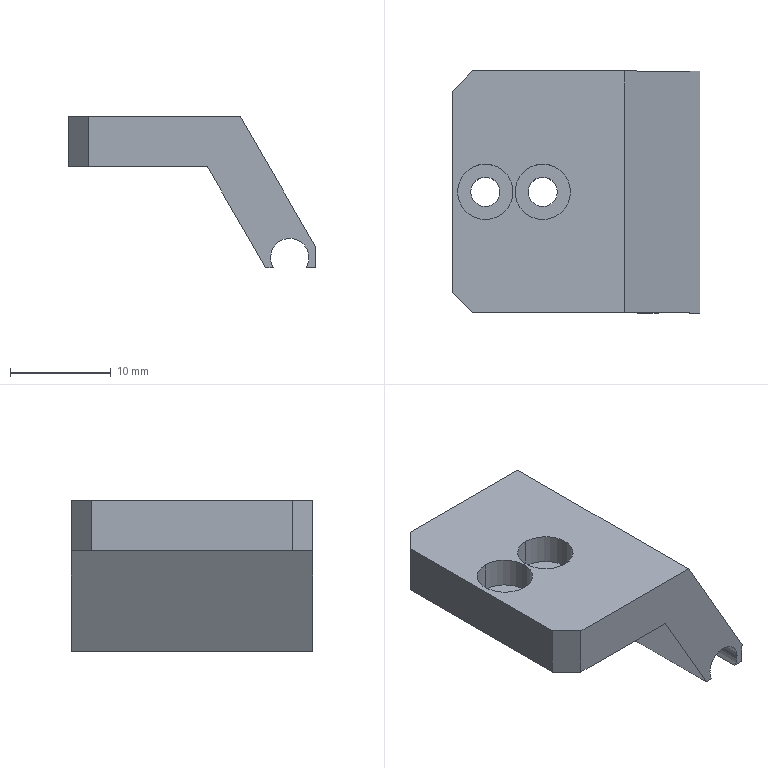Component | SolidWorks | 31298300012MechanicalFinger-1 | 1 solid | 25 faces | box 24.6 x 24 x 15 mm | volume 3262 mm3 | plane 14 | cylinder 11 | commonest cylinder face diameters 5.5 x4 2.9 x4 3.8 x3 | material Q235-A
build123d program:
from build123d import *

# Parameters (mm, degrees)
BOSS_EXTRUDE1_DEPTH                               = 12
M2_5_HEX_SOCKET_HEAD_CAP_SCREW_CBORE1_D           = 2.9
M2_5_HEX_SOCKET_HEAD_CAP_SCREW_CBORE1_CBORE_D     = 5.5
M2_5_HEX_SOCKET_HEAD_CAP_SCREW_CBORE1_CBORE_DEPTH = 3
CHAMFER1_SIZE                                     = 2
SKETCH5_R                                         = 1.9
CUT_EXTRUDE2_DEPTH                                = 38.499


with BuildPart() as part:
    # Sketch1 → Boss-Extrude1 (new, symmetric)
    with BuildSketch(Plane.XY):
        Polygon((0, 0), (17.094, 0), (24.6, -13), (24.6, -15), (19.6, -15), (13.826, -5), (0, -5), align=None)
    extrude(amount=BOSS_EXTRUDE1_DEPTH, both=True)

    # M2.5 Hex Socket Head Cap Screw CBORE1 (through all)
    with Locations(Plane(origin=(0, 0, 0), x_dir=(-1, 0, 0), z_dir=(0, 1, 0))):
        with Locations((-3.3, 0), (-9, 0)):
            CounterBoreHole(M2_5_HEX_SOCKET_HEAD_CAP_SCREW_CBORE1_D / 2, M2_5_HEX_SOCKET_HEAD_CAP_SCREW_CBORE1_CBORE_D / 2, M2_5_HEX_SOCKET_HEAD_CAP_SCREW_CBORE1_CBORE_DEPTH)

    # Chamfer1
    chamfer1_edges = [part.edges().sort_by_distance(p)[0] for p in [
        (0, -2.5, 12),
        (0, -2.5, -12),
    ]]
    chamfer(chamfer1_edges, length=CHAMFER1_SIZE)

    # Sketch5 → Cut-Extrude2 (cut, through all)
    with BuildSketch(Plane.XY.offset(12)):
        with Locations((22, -14)):
            Circle(SKETCH5_R)
    extrude(amount=-CUT_EXTRUDE2_DEPTH, mode=Mode.SUBTRACT)


solid = part.part

# Placed as in the assembly
solid = solid.moved(Location((188.87, 43.668, 52.929), (90, 0, 0)))
STEP:
#1=COLOUR_RGB('',0.7922,0.8196,0.9333);
#2=FILL_AREA_STYLE_COLOUR('',#1);
#3=FILL_AREA_STYLE('',(#2));
#4=SURFACE_STYLE_FILL_AREA(#3);
#5=SURFACE_SIDE_STYLE('',(#4));
#6=SURFACE_STYLE_USAGE(.BOTH.,#5);
#7=PRESENTATION_STYLE_ASSIGNMENT((#6));
#8=CARTESIAN_POINT('',(8.238,2.192,1.493));
#9=VERTEX_POINT('',#8);
#10=CARTESIAN_POINT('',(8.227,2.192,1.533));
#11=VERTEX_POINT('',#10);
#12=CARTESIAN_POINT('',(8.302,2.192,1.533));
#13=DIRECTION('',(-0.,1.,-0.));
#14=DIRECTION('',(-1.,0.,0.));
#15=AXIS2_PLACEMENT_3D('',#12,#13,#14);
#16=CIRCLE('',#15,0.0748);
#17=EDGE_CURVE('',#9,#11,#16,.T.);
#18=ORIENTED_EDGE('',*,*,#17,.T.);
#19=CARTESIAN_POINT('',(8.227,1.247,1.533));
#20=VERTEX_POINT('',#19);
#21=CARTESIAN_POINT('',(8.227,2.192,1.533));
#22=DIRECTION('',(0.,-1.,0.));
#23=VECTOR('',#22,39.37);
#24=LINE('',#21,#23);
#25=EDGE_CURVE('',#11,#20,#24,.T.);
#26=ORIENTED_EDGE('',*,*,#25,.T.);
#27=CARTESIAN_POINT('',(8.238,1.247,1.493));
#28=VERTEX_POINT('',#27);
#29=CARTESIAN_POINT('',(8.302,1.247,1.533));
#30=DIRECTION('',(0.,-1.,0.));
#31=DIRECTION('',(1.,0.,0.));
#32=AXIS2_PLACEMENT_3D('',#29,#30,#31);
#33=CIRCLE('',#32,0.0748);
#34=EDGE_CURVE('',#20,#28,#33,.T.);
#35=ORIENTED_EDGE('',*,*,#34,.T.);
#36=CARTESIAN_POINT('',(8.238,2.192,1.493));
#37=DIRECTION('',(0.,-1.,0.));
#38=VECTOR('',#37,39.37);
#39=LINE('',#36,#38);
#40=EDGE_CURVE('',#9,#28,#39,.T.);
#41=ORIENTED_EDGE('',*,*,#40,.F.);
#42=EDGE_LOOP('',(#18,#26,#35,#41));
#43=FACE_OUTER_BOUND('',#42,.T.);
#44=CARTESIAN_POINT('',(8.302,2.192,1.533));
#45=DIRECTION('',(0.,-1.,0.));
#46=DIRECTION('',(1.,0.,0.));
#47=AXIS2_PLACEMENT_3D('',#44,#45,#46);
#48=CYLINDRICAL_SURFACE('',#47,0.0748);
#49=ADVANCED_FACE('',(#43),#48,.F.);
#50=ORIENTED_EDGE('',*,*,#25,.F.);
#51=CARTESIAN_POINT('',(8.377,2.192,1.533));
#52=VERTEX_POINT('',#51);
#53=CARTESIAN_POINT('',(8.302,2.192,1.533));
#54=DIRECTION('',(-0.,1.,-0.));
#55=DIRECTION('',(-1.,0.,0.));
#56=AXIS2_PLACEMENT_3D('',#53,#54,#55);
#57=CIRCLE('',#56,0.0748);
#58=EDGE_CURVE('',#11,#52,#57,.T.);
#59=ORIENTED_EDGE('',*,*,#58,.T.);
#60=CARTESIAN_POINT('',(8.377,1.247,1.533));
#61=VERTEX_POINT('',#60);
#62=CARTESIAN_POINT('',(8.377,2.192,1.533));
#63=DIRECTION('',(0.,-1.,0.));
#64=VECTOR('',#63,39.37);
#65=LINE('',#62,#64);
#66=EDGE_CURVE('',#52,#61,#65,.T.);
#67=ORIENTED_EDGE('',*,*,#66,.T.);
#68=CARTESIAN_POINT('',(8.302,1.247,1.533));
#69=DIRECTION('',(0.,-1.,0.));
#70=DIRECTION('',(1.,0.,0.));
#71=AXIS2_PLACEMENT_3D('',#68,#69,#70);
#72=CIRCLE('',#71,0.0748);
#73=EDGE_CURVE('',#61,#20,#72,.T.);
#74=ORIENTED_EDGE('',*,*,#73,.T.);
#75=EDGE_LOOP('',(#50,#59,#67,#74));
#76=FACE_OUTER_BOUND('',#75,.T.);
#77=CARTESIAN_POINT('',(8.302,2.192,1.533));
#78=DIRECTION('',(0.,-1.,0.));
#79=DIRECTION('',(1.,0.,0.));
#80=AXIS2_PLACEMENT_3D('',#77,#78,#79);
#81=CYLINDRICAL_SURFACE('',#80,0.0748);
#82=ADVANCED_FACE('',(#76),#81,.F.);
#83=CARTESIAN_POINT('',(7.566,1.827,1.966));
#84=VERTEX_POINT('',#83);
#85=CARTESIAN_POINT('',(7.566,1.611,1.966));
#86=VERTEX_POINT('',#85);
#87=CARTESIAN_POINT('',(7.566,1.719,1.966));
#88=DIRECTION('',(0.,0.,1.));
#89=DIRECTION('',(0.,-1.,0.));
#90=AXIS2_PLACEMENT_3D('',#87,#88,#89);
#91=CIRCLE('',#90,0.1083);
#92=EDGE_CURVE('',#84,#86,#91,.T.);
#93=ORIENTED_EDGE('',*,*,#92,.F.);
#94=CARTESIAN_POINT('',(7.566,1.827,2.084));
#95=VERTEX_POINT('',#94);
#96=CARTESIAN_POINT('',(7.566,1.827,2.084));
#97=DIRECTION('',(0.,0.,1.));
#98=VECTOR('',#97,39.37);
#99=LINE('',#96,#98);
#100=EDGE_CURVE('',#84,#95,#99,.T.);
#101=ORIENTED_EDGE('',*,*,#100,.T.);
#102=CARTESIAN_POINT('',(7.566,1.611,2.084));
#103=VERTEX_POINT('',#102);
#104=CARTESIAN_POINT('',(7.566,1.719,2.084));
#105=DIRECTION('',(0.,0.,1.));
#106=DIRECTION('',(0.,-1.,0.));
#107=AXIS2_PLACEMENT_3D('',#104,#105,#106);
#108=CIRCLE('',#107,0.1083);
#109=EDGE_CURVE('',#95,#103,#108,.T.);
#110=ORIENTED_EDGE('',*,*,#109,.T.);
#111=CARTESIAN_POINT('',(7.566,1.611,2.084));
#112=DIRECTION('',(0.,0.,1.));
#113=VECTOR('',#112,39.37);
#114=LINE('',#111,#113);
#115=EDGE_CURVE('',#86,#103,#114,.T.);
#116=ORIENTED_EDGE('',*,*,#115,.F.);
#117=EDGE_LOOP('',(#93,#101,#110,#116));
#118=FACE_OUTER_BOUND('',#117,.T.);
#119=CARTESIAN_POINT('',(7.566,1.719,2.084));
#120=DIRECTION('',(0.,0.,1.));
#121=DIRECTION('',(0.,-1.,0.));
#122=AXIS2_PLACEMENT_3D('',#119,#120,#121);
#123=CYLINDRICAL_SURFACE('',#122,0.1083);
#124=ADVANCED_FACE('',(#118),#123,.F.);
#125=CARTESIAN_POINT('',(7.566,1.776,1.887));
#126=VERTEX_POINT('',#125);
#127=CARTESIAN_POINT('',(7.566,1.662,1.887));
#128=VERTEX_POINT('',#127);
#129=CARTESIAN_POINT('',(7.566,1.719,1.887));
#130=DIRECTION('',(0.,0.,1.));
#131=DIRECTION('',(-1.,0.,0.));
#132=AXIS2_PLACEMENT_3D('',#129,#130,#131);
#133=CIRCLE('',#132,0.05709);
#134=EDGE_CURVE('',#126,#128,#133,.T.);
#135=ORIENTED_EDGE('',*,*,#134,.F.);
#136=CARTESIAN_POINT('',(7.566,1.776,1.966));
#137=VERTEX_POINT('',#136);
#138=CARTESIAN_POINT('',(7.566,1.776,2.084));
#139=DIRECTION('',(0.,0.,1.));
#140=VECTOR('',#139,39.37);
#141=LINE('',#138,#140);
#142=EDGE_CURVE('',#126,#137,#141,.T.);
#143=ORIENTED_EDGE('',*,*,#142,.T.);
#144=CARTESIAN_POINT('',(7.566,1.662,1.966));
#145=VERTEX_POINT('',#144);
#146=CARTESIAN_POINT('',(7.566,1.719,1.966));
#147=DIRECTION('',(0.,0.,1.));
#148=DIRECTION('',(0.,-1.,0.));
#149=AXIS2_PLACEMENT_3D('',#146,#147,#148);
#150=CIRCLE('',#149,0.05709);
#151=EDGE_CURVE('',#137,#145,#150,.T.);
#152=ORIENTED_EDGE('',*,*,#151,.T.);
#153=CARTESIAN_POINT('',(7.566,1.662,2.084));
#154=DIRECTION('',(0.,0.,1.));
#155=VECTOR('',#154,39.37);
#156=LINE('',#153,#155);
#157=EDGE_CURVE('',#128,#145,#156,.T.);
#158=ORIENTED_EDGE('',*,*,#157,.F.);
#159=EDGE_LOOP('',(#135,#143,#152,#158));
#160=FACE_OUTER_BOUND('',#159,.T.);
#161=CARTESIAN_POINT('',(7.566,1.719,2.084));
#162=DIRECTION('',(0.,0.,1.));
#163=DIRECTION('',(0.,-1.,0.));
#164=AXIS2_PLACEMENT_3D('',#161,#162,#163);
#165=CYLINDRICAL_SURFACE('',#164,0.05709);
#166=ADVANCED_FACE('',(#160),#165,.F.);
#167=CARTESIAN_POINT('',(7.79,1.827,1.966));
#168=VERTEX_POINT('',#167);
#169=CARTESIAN_POINT('',(7.79,1.611,1.966));
#170=VERTEX_POINT('',#169);
#171=CARTESIAN_POINT('',(7.79,1.719,1.966));
#172=DIRECTION('',(0.,0.,1.));
#173=DIRECTION('',(0.,-1.,0.));
#174=AXIS2_PLACEMENT_3D('',#171,#172,#173);
#175=CIRCLE('',#174,0.1083);
#176=EDGE_CURVE('',#168,#170,#175,.T.);
#177=ORIENTED_EDGE('',*,*,#176,.F.);
#178=CARTESIAN_POINT('',(7.79,1.827,2.084));
#179=VERTEX_POINT('',#178);
#180=CARTESIAN_POINT('',(7.79,1.827,2.084));
#181=DIRECTION('',(0.,0.,1.));
#182=VECTOR('',#181,39.37);
#183=LINE('',#180,#182);
#184=EDGE_CURVE('',#168,#179,#183,.T.);
#185=ORIENTED_EDGE('',*,*,#184,.T.);
#186=CARTESIAN_POINT('',(7.79,1.611,2.084));
#187=VERTEX_POINT('',#186);
#188=CARTESIAN_POINT('',(7.79,1.719,2.084));
#189=DIRECTION('',(0.,0.,1.));
#190=DIRECTION('',(0.,-1.,0.));
#191=AXIS2_PLACEMENT_3D('',#188,#189,#190);
#192=CIRCLE('',#191,0.1083);
#193=EDGE_CURVE('',#179,#187,#192,.T.);
#194=ORIENTED_EDGE('',*,*,#193,.T.);
#195=CARTESIAN_POINT('',(7.79,1.611,2.084));
#196=DIRECTION('',(0.,0.,1.));
#197=VECTOR('',#196,39.37);
#198=LINE('',#195,#197);
#199=EDGE_CURVE('',#170,#187,#198,.T.);
#200=ORIENTED_EDGE('',*,*,#199,.F.);
#201=EDGE_LOOP('',(#177,#185,#194,#200));
#202=FACE_OUTER_BOUND('',#201,.T.);
#203=CARTESIAN_POINT('',(7.79,1.719,2.084));
#204=DIRECTION('',(0.,0.,1.));
#205=DIRECTION('',(0.,-1.,0.));
#206=AXIS2_PLACEMENT_3D('',#203,#204,#205);
#207=CYLINDRICAL_SURFACE('',#206,0.1083);
#208=ADVANCED_FACE('',(#202),#207,.F.);
#209=CARTESIAN_POINT('',(7.79,1.776,1.887));
#210=VERTEX_POINT('',#209);
#211=CARTESIAN_POINT('',(7.79,1.662,1.887));
#212=VERTEX_POINT('',#211);
#213=CARTESIAN_POINT('',(7.79,1.719,1.887));
#214=DIRECTION('',(0.,0.,1.));
#215=DIRECTION('',(-1.,0.,0.));
#216=AXIS2_PLACEMENT_3D('',#213,#214,#215);
#217=CIRCLE('',#216,0.05709);
#218=EDGE_CURVE('',#210,#212,#217,.T.);
#219=ORIENTED_EDGE('',*,*,#218,.F.);
#220=CARTESIAN_POINT('',(7.79,1.776,1.966));
#221=VERTEX_POINT('',#220);
#222=CARTESIAN_POINT('',(7.79,1.776,2.084));
#223=DIRECTION('',(0.,0.,1.));
#224=VECTOR('',#223,39.37);
#225=LINE('',#222,#224);
#226=EDGE_CURVE('',#210,#221,#225,.T.);
#227=ORIENTED_EDGE('',*,*,#226,.T.);
#228=CARTESIAN_POINT('',(7.79,1.662,1.966));
#229=VERTEX_POINT('',#228);
#230=CARTESIAN_POINT('',(7.79,1.719,1.966));
#231=DIRECTION('',(0.,0.,1.));
#232=DIRECTION('',(0.,-1.,0.));
#233=AXIS2_PLACEMENT_3D('',#230,#231,#232);
#234=CIRCLE('',#233,0.05709);
#235=EDGE_CURVE('',#221,#229,#234,.T.);
#236=ORIENTED_EDGE('',*,*,#235,.T.);
#237=CARTESIAN_POINT('',(7.79,1.662,2.084));
#238=DIRECTION('',(0.,0.,1.));
#239=VECTOR('',#238,39.37);
#240=LINE('',#237,#239);
#241=EDGE_CURVE('',#212,#229,#240,.T.);
#242=ORIENTED_EDGE('',*,*,#241,.F.);
#243=EDGE_LOOP('',(#219,#227,#236,#242));
#244=FACE_OUTER_BOUND('',#243,.T.);
#245=CARTESIAN_POINT('',(7.79,1.719,2.084));
#246=DIRECTION('',(0.,0.,1.));
#247=DIRECTION('',(0.,-1.,0.));
#248=AXIS2_PLACEMENT_3D('',#245,#246,#247);
#249=CYLINDRICAL_SURFACE('',#248,0.05709);
#250=ADVANCED_FACE('',(#244),#249,.F.);
#251=CARTESIAN_POINT('',(8.207,2.192,1.493));
#252=VERTEX_POINT('',#251);
#253=CARTESIAN_POINT('',(8.404,2.192,1.493));
#254=DIRECTION('',(1.,0.,-0.));
#255=VECTOR('',#254,39.37);
#256=LINE('',#253,#255);
#257=EDGE_CURVE('',#252,#9,#256,.T.);
#258=ORIENTED_EDGE('',*,*,#257,.T.);
#259=ORIENTED_EDGE('',*,*,#40,.T.);
#260=CARTESIAN_POINT('',(8.207,1.247,1.493));
#261=VERTEX_POINT('',#260);
#262=CARTESIAN_POINT('',(8.404,1.247,1.493));
#263=DIRECTION('',(1.,0.,-0.));
#264=VECTOR('',#263,39.37);
#265=LINE('',#262,#264);
#266=EDGE_CURVE('',#261,#28,#265,.T.);
#267=ORIENTED_EDGE('',*,*,#266,.F.);
#268=CARTESIAN_POINT('',(8.207,1.247,1.493));
#269=DIRECTION('',(-0.,1.,-0.));
#270=VECTOR('',#269,39.37);
#271=LINE('',#268,#270);
#272=EDGE_CURVE('',#261,#252,#271,.T.);
#273=ORIENTED_EDGE('',*,*,#272,.T.);
#274=EDGE_LOOP('',(#258,#259,#267,#273));
#275=FACE_OUTER_BOUND('',#274,.T.);
#276=CARTESIAN_POINT('',(8.404,1.247,1.493));
#277=DIRECTION('',(0.,0.,1.));
#278=DIRECTION('',(0.,-1.,0.));
#279=AXIS2_PLACEMENT_3D('',#276,#277,#278);
#280=PLANE('',#279);
#281=ADVANCED_FACE('',(#275),#280,.F.);
#282=CARTESIAN_POINT('',(7.436,1.326,1.887));
#283=VERTEX_POINT('',#282);
#284=CARTESIAN_POINT('',(7.436,2.113,1.887));
#285=VERTEX_POINT('',#284);
#286=CARTESIAN_POINT('',(7.436,1.247,1.887));
#287=DIRECTION('',(-0.,1.,-0.));
#288=VECTOR('',#287,39.37);
#289=LINE('',#286,#288);
#290=EDGE_CURVE('',#283,#285,#289,.T.);
#291=ORIENTED_EDGE('',*,*,#290,.F.);
#292=CARTESIAN_POINT('',(7.436,1.326,2.084));
#293=VERTEX_POINT('',#292);
#294=CARTESIAN_POINT('',(7.436,1.326,1.887));
#295=DIRECTION('',(0.,0.,1.));
#296=VECTOR('',#295,39.37);
#297=LINE('',#294,#296);
#298=EDGE_CURVE('',#283,#293,#297,.T.);
#299=ORIENTED_EDGE('',*,*,#298,.T.);
#300=CARTESIAN_POINT('',(7.436,2.113,2.084));
#301=VERTEX_POINT('',#300);
#302=CARTESIAN_POINT('',(7.436,1.247,2.084));
#303=DIRECTION('',(-0.,1.,-0.));
#304=VECTOR('',#303,39.37);
#305=LINE('',#302,#304);
#306=EDGE_CURVE('',#293,#301,#305,.T.);
#307=ORIENTED_EDGE('',*,*,#306,.T.);
#308=CARTESIAN_POINT('',(7.436,2.113,1.887));
#309=DIRECTION('',(-0.,-0.,-1.));
#310=VECTOR('',#309,39.37);
#311=LINE('',#308,#310);
#312=EDGE_CURVE('',#301,#285,#311,.T.);
#313=ORIENTED_EDGE('',*,*,#312,.T.);
#314=EDGE_LOOP('',(#291,#299,#307,#313));
#315=FACE_OUTER_BOUND('',#314,.T.);
#316=CARTESIAN_POINT('',(7.436,1.247,1.887));
#317=DIRECTION('',(1.,0.,-0.));
#318=DIRECTION('',(-0.,1.,-0.));
#319=AXIS2_PLACEMENT_3D('',#316,#317,#318);
#320=PLANE('',#319);
#321=ADVANCED_FACE('',(#315),#320,.F.);
#322=CARTESIAN_POINT('',(7.566,1.719,1.887));
#323=DIRECTION('',(0.,0.,1.));
#324=DIRECTION('',(-1.,0.,0.));
#325=AXIS2_PLACEMENT_3D('',#322,#323,#324);
#326=CIRCLE('',#325,0.05709);
#327=EDGE_CURVE('',#128,#126,#326,.T.);
#328=ORIENTED_EDGE('',*,*,#327,.T.);
#329=ORIENTED_EDGE('',*,*,#134,.T.);
#330=EDGE_LOOP('',(#328,#329));
#331=FACE_BOUND('',#330,.T.);
#332=CARTESIAN_POINT('',(7.79,1.719,1.887));
#333=DIRECTION('',(0.,0.,1.));
#334=DIRECTION('',(-1.,0.,0.));
#335=AXIS2_PLACEMENT_3D('',#332,#333,#334);
#336=CIRCLE('',#335,0.05709);
#337=EDGE_CURVE('',#212,#210,#336,.T.);
#338=ORIENTED_EDGE('',*,*,#337,.T.);
#339=ORIENTED_EDGE('',*,*,#218,.T.);
#340=EDGE_LOOP('',(#338,#339));
#341=FACE_BOUND('',#340,.T.);
#342=CARTESIAN_POINT('',(7.515,1.247,1.887));
#343=VERTEX_POINT('',#342);
#344=CARTESIAN_POINT('',(7.98,1.247,1.887));
#345=VERTEX_POINT('',#344);
#346=CARTESIAN_POINT('',(7.98,1.247,1.887));
#347=DIRECTION('',(1.,0.,-0.));
#348=VECTOR('',#347,39.37);
#349=LINE('',#346,#348);
#350=EDGE_CURVE('',#343,#345,#349,.T.);
#351=ORIENTED_EDGE('',*,*,#350,.F.);
#352=CARTESIAN_POINT('',(7.515,1.247,1.887));
#353=DIRECTION('',(-0.7071,0.7071,0.));
#354=VECTOR('',#353,39.37);
#355=LINE('',#352,#354);
#356=EDGE_CURVE('',#343,#283,#355,.T.);
#357=ORIENTED_EDGE('',*,*,#356,.T.);
#358=ORIENTED_EDGE('',*,*,#290,.T.);
#359=CARTESIAN_POINT('',(7.515,2.192,1.887));
#360=VERTEX_POINT('',#359);
#361=CARTESIAN_POINT('',(7.436,2.113,1.887));
#362=DIRECTION('',(0.7071,0.7071,-0.));
#363=VECTOR('',#362,39.37);
#364=LINE('',#361,#363);
#365=EDGE_CURVE('',#285,#360,#364,.T.);
#366=ORIENTED_EDGE('',*,*,#365,.T.);
#367=CARTESIAN_POINT('',(7.98,2.192,1.887));
#368=VERTEX_POINT('',#367);
#369=CARTESIAN_POINT('',(7.98,2.192,1.887));
#370=DIRECTION('',(1.,0.,-0.));
#371=VECTOR('',#370,39.37);
#372=LINE('',#369,#371);
#373=EDGE_CURVE('',#360,#368,#372,.T.);
#374=ORIENTED_EDGE('',*,*,#373,.T.);
#375=CARTESIAN_POINT('',(7.98,1.247,1.887));
#376=DIRECTION('',(-0.,1.,-0.));
#377=VECTOR('',#376,39.37);
#378=LINE('',#375,#377);
#379=EDGE_CURVE('',#345,#368,#378,.T.);
#380=ORIENTED_EDGE('',*,*,#379,.F.);
#381=EDGE_LOOP('',(#351,#357,#358,#366,#374,#380));
#382=FACE_OUTER_BOUND('',#381,.T.);
#383=CARTESIAN_POINT('',(7.98,1.247,1.887));
#384=DIRECTION('',(0.,0.,1.));
#385=DIRECTION('',(-1.,-0.,0.));
#386=AXIS2_PLACEMENT_3D('',#383,#384,#385);
#387=PLANE('',#386);
#388=ADVANCED_FACE('',(#331,#341,#382),#387,.F.);
#389=CARTESIAN_POINT('',(8.207,2.192,1.493));
#390=DIRECTION('',(0.5,0.,-0.866));
#391=VECTOR('',#390,39.37);
#392=LINE('',#389,#391);
#393=EDGE_CURVE('',#368,#252,#392,.T.);
#394=ORIENTED_EDGE('',*,*,#393,.T.);
#395=ORIENTED_EDGE('',*,*,#272,.F.);
#396=CARTESIAN_POINT('',(8.207,1.247,1.493));
#397=DIRECTION('',(0.5,0.,-0.866));
#398=VECTOR('',#397,39.37);
#399=LINE('',#396,#398);
#400=EDGE_CURVE('',#345,#261,#399,.T.);
#401=ORIENTED_EDGE('',*,*,#400,.F.);
#402=ORIENTED_EDGE('',*,*,#379,.T.);
#403=EDGE_LOOP('',(#394,#395,#401,#402));
#404=FACE_OUTER_BOUND('',#403,.T.);
#405=CARTESIAN_POINT('',(8.207,1.247,1.493));
#406=DIRECTION('',(0.866,0.,0.5));
#407=DIRECTION('',(-0.5,-0.,0.866));
#408=AXIS2_PLACEMENT_3D('',#405,#406,#407);
#409=PLANE('',#408);
#410=ADVANCED_FACE('',(#404),#409,.F.);
#411=CARTESIAN_POINT('',(8.366,1.247,1.493));
#412=VERTEX_POINT('',#411);
#413=CARTESIAN_POINT('',(8.404,1.247,1.493));
#414=VERTEX_POINT('',#413);
#415=CARTESIAN_POINT('',(8.404,1.247,1.493));
#416=DIRECTION('',(1.,0.,-0.));
#417=VECTOR('',#416,39.37);
#418=LINE('',#415,#417);
#419=EDGE_CURVE('',#412,#414,#418,.T.);
#420=ORIENTED_EDGE('',*,*,#419,.F.);
#421=CARTESIAN_POINT('',(8.366,2.192,1.493));
#422=VERTEX_POINT('',#421);
#423=CARTESIAN_POINT('',(8.366,2.192,1.493));
#424=DIRECTION('',(-0.,1.,-0.));
#425=VECTOR('',#424,39.37);
#426=LINE('',#423,#425);
#427=EDGE_CURVE('',#412,#422,#426,.T.);
#428=ORIENTED_EDGE('',*,*,#427,.T.);
#429=CARTESIAN_POINT('',(8.404,2.192,1.493));
#430=VERTEX_POINT('',#429);
#431=CARTESIAN_POINT('',(8.404,2.192,1.493));
#432=DIRECTION('',(1.,0.,-0.));
#433=VECTOR('',#432,39.37);
#434=LINE('',#431,#433);
#435=EDGE_CURVE('',#422,#430,#434,.T.);
#436=ORIENTED_EDGE('',*,*,#435,.T.);
#437=CARTESIAN_POINT('',(8.404,1.247,1.493));
#438=DIRECTION('',(-0.,1.,-0.));
#439=VECTOR('',#438,39.37);
#440=LINE('',#437,#439);
#441=EDGE_CURVE('',#414,#430,#440,.T.);
#442=ORIENTED_EDGE('',*,*,#441,.F.);
#443=EDGE_LOOP('',(#420,#428,#436,#442));
#444=FACE_OUTER_BOUND('',#443,.T.);
#445=CARTESIAN_POINT('',(8.404,1.247,1.493));
#446=DIRECTION('',(0.,0.,1.));
#447=DIRECTION('',(0.,-1.,0.));
#448=AXIS2_PLACEMENT_3D('',#445,#446,#447);
#449=PLANE('',#448);
#450=ADVANCED_FACE('',(#444),#449,.F.);
#451=CARTESIAN_POINT('',(8.404,2.192,1.572));
#452=VERTEX_POINT('',#451);
#453=CARTESIAN_POINT('',(8.404,2.192,1.572));
#454=DIRECTION('',(0.,0.,1.));
#455=VECTOR('',#454,39.37);
#456=LINE('',#453,#455);
#457=EDGE_CURVE('',#430,#452,#456,.T.);
#458=ORIENTED_EDGE('',*,*,#457,.T.);
#459=CARTESIAN_POINT('',(8.404,1.247,1.572));
#460=VERTEX_POINT('',#459);
#461=CARTESIAN_POINT('',(8.404,1.247,1.572));
#462=DIRECTION('',(-0.,1.,-0.));
#463=VECTOR('',#462,39.37);
#464=LINE('',#461,#463);
#465=EDGE_CURVE('',#460,#452,#464,.T.);
#466=ORIENTED_EDGE('',*,*,#465,.F.);
#467=CARTESIAN_POINT('',(8.404,1.247,1.572));
#468=DIRECTION('',(0.,0.,1.));
#469=VECTOR('',#468,39.37);
#470=LINE('',#467,#469);
#471=EDGE_CURVE('',#414,#460,#470,.T.);
#472=ORIENTED_EDGE('',*,*,#471,.F.);
#473=ORIENTED_EDGE('',*,*,#441,.T.);
#474=EDGE_LOOP('',(#458,#466,#472,#473));
#475=FACE_OUTER_BOUND('',#474,.T.);
#476=CARTESIAN_POINT('',(8.404,1.247,1.572));
#477=DIRECTION('',(-1.,-0.,0.));
#478=DIRECTION('',(0.,-1.,0.));
#479=AXIS2_PLACEMENT_3D('',#476,#477,#478);
#480=PLANE('',#479);
#481=ADVANCED_FACE('',(#475),#480,.F.);
#482=CARTESIAN_POINT('',(8.109,2.192,2.084));
#483=VERTEX_POINT('',#482);
#484=CARTESIAN_POINT('',(8.109,2.192,2.084));
#485=DIRECTION('',(-0.5,-0.,0.866));
#486=VECTOR('',#485,39.37);
#487=LINE('',#484,#486);
#488=EDGE_CURVE('',#452,#483,#487,.T.);
#489=ORIENTED_EDGE('',*,*,#488,.T.);
#490=CARTESIAN_POINT('',(8.109,1.247,2.084));
#491=VERTEX_POINT('',#490);
#492=CARTESIAN_POINT('',(8.109,1.247,2.084));
#493=DIRECTION('',(-0.,1.,-0.));
#494=VECTOR('',#493,39.37);
#495=LINE('',#492,#494);
#496=EDGE_CURVE('',#491,#483,#495,.T.);
#497=ORIENTED_EDGE('',*,*,#496,.F.);
#498=CARTESIAN_POINT('',(8.109,1.247,2.084));
#499=DIRECTION('',(-0.5,-0.,0.866));
#500=VECTOR('',#499,39.37);
#501=LINE('',#498,#500);
#502=EDGE_CURVE('',#460,#491,#501,.T.);
#503=ORIENTED_EDGE('',*,*,#502,.F.);
#504=ORIENTED_EDGE('',*,*,#465,.T.);
#505=EDGE_LOOP('',(#489,#497,#503,#504));
#506=FACE_OUTER_BOUND('',#505,.T.);
#507=CARTESIAN_POINT('',(8.109,1.247,2.084));
#508=DIRECTION('',(-0.866,-0.,-0.5));
#509=DIRECTION('',(0.5,0.,-0.866));
#510=AXIS2_PLACEMENT_3D('',#507,#508,#509);
#511=PLANE('',#510);
#512=ADVANCED_FACE('',(#506),#511,.F.);
#513=CARTESIAN_POINT('',(7.566,1.719,2.084));
#514=DIRECTION('',(0.,0.,1.));
#515=DIRECTION('',(0.,-1.,0.));
#516=AXIS2_PLACEMENT_3D('',#513,#514,#515);
#517=CIRCLE('',#516,0.1083);
#518=EDGE_CURVE('',#103,#95,#517,.T.);
#519=ORIENTED_EDGE('',*,*,#518,.F.);
#520=ORIENTED_EDGE('',*,*,#109,.F.);
#521=EDGE_LOOP('',(#519,#520));
#522=FACE_BOUND('',#521,.T.);
#523=CARTESIAN_POINT('',(7.79,1.719,2.084));
#524=DIRECTION('',(0.,0.,1.));
#525=DIRECTION('',(0.,-1.,0.));
#526=AXIS2_PLACEMENT_3D('',#523,#524,#525);
#527=CIRCLE('',#526,0.1083);
#528=EDGE_CURVE('',#187,#179,#527,.T.);
#529=ORIENTED_EDGE('',*,*,#528,.F.);
#530=ORIENTED_EDGE('',*,*,#193,.F.);
#531=EDGE_LOOP('',(#529,#530));
#532=FACE_BOUND('',#531,.T.);
#533=ORIENTED_EDGE('',*,*,#306,.F.);
#534=CARTESIAN_POINT('',(7.515,1.247,2.084));
#535=VERTEX_POINT('',#534);
#536=CARTESIAN_POINT('',(7.515,1.247,2.084));
#537=DIRECTION('',(0.7071,-0.7071,-0.));
#538=VECTOR('',#537,39.37);
#539=LINE('',#536,#538);
#540=EDGE_CURVE('',#293,#535,#539,.T.);
#541=ORIENTED_EDGE('',*,*,#540,.T.);
#542=CARTESIAN_POINT('',(7.436,1.247,2.084));
#543=DIRECTION('',(-1.,-0.,0.));
#544=VECTOR('',#543,39.37);
#545=LINE('',#542,#544);
#546=EDGE_CURVE('',#491,#535,#545,.T.);
#547=ORIENTED_EDGE('',*,*,#546,.F.);
#548=ORIENTED_EDGE('',*,*,#496,.T.);
#549=CARTESIAN_POINT('',(7.515,2.192,2.084));
#550=VERTEX_POINT('',#549);
#551=CARTESIAN_POINT('',(7.436,2.192,2.084));
#552=DIRECTION('',(-1.,-0.,0.));
#553=VECTOR('',#552,39.37);
#554=LINE('',#551,#553);
#555=EDGE_CURVE('',#483,#550,#554,.T.);
#556=ORIENTED_EDGE('',*,*,#555,.T.);
#557=CARTESIAN_POINT('',(7.436,2.113,2.084));
#558=DIRECTION('',(-0.7071,-0.7071,0.));
#559=VECTOR('',#558,39.37);
#560=LINE('',#557,#559);
#561=EDGE_CURVE('',#550,#301,#560,.T.);
#562=ORIENTED_EDGE('',*,*,#561,.T.);
#563=EDGE_LOOP('',(#533,#541,#547,#548,#556,#562));
#564=FACE_OUTER_BOUND('',#563,.T.);
#565=CARTESIAN_POINT('',(7.436,1.247,2.084));
#566=DIRECTION('',(-0.,-0.,-1.));
#567=DIRECTION('',(-0.,1.,-0.));
#568=AXIS2_PLACEMENT_3D('',#565,#566,#567);
#569=PLANE('',#568);
#570=ADVANCED_FACE('',(#522,#532,#564),#569,.F.);
#571=ORIENTED_EDGE('',*,*,#266,.T.);
#572=ORIENTED_EDGE('',*,*,#34,.F.);
#573=ORIENTED_EDGE('',*,*,#73,.F.);
#574=CARTESIAN_POINT('',(8.302,1.247,1.533));
#575=DIRECTION('',(0.,-1.,0.));
#576=DIRECTION('',(1.,0.,0.));
#577=AXIS2_PLACEMENT_3D('',#574,#575,#576);
#578=CIRCLE('',#577,0.0748);
#579=EDGE_CURVE('',#412,#61,#578,.T.);
#580=ORIENTED_EDGE('',*,*,#579,.F.);
#581=ORIENTED_EDGE('',*,*,#419,.T.);
#582=ORIENTED_EDGE('',*,*,#471,.T.);
#583=ORIENTED_EDGE('',*,*,#502,.T.);
#584=ORIENTED_EDGE('',*,*,#546,.T.);
#585=CARTESIAN_POINT('',(7.515,1.247,2.084));
#586=DIRECTION('',(-0.,-0.,-1.));
#587=VECTOR('',#586,39.37);
#588=LINE('',#585,#587);
#589=EDGE_CURVE('',#535,#343,#588,.T.);
#590=ORIENTED_EDGE('',*,*,#589,.T.);
#591=ORIENTED_EDGE('',*,*,#350,.T.);
#592=ORIENTED_EDGE('',*,*,#400,.T.);
#593=EDGE_LOOP('',(#571,#572,#573,#580,#581,#582,#583,#584,#590,#591,#592));
#594=FACE_OUTER_BOUND('',#593,.T.);
#595=CARTESIAN_POINT('',(7.436,1.247,2.084));
#596=DIRECTION('',(-0.,1.,-0.));
#597=DIRECTION('',(-1.,-0.,0.));
#598=AXIS2_PLACEMENT_3D('',#595,#596,#597);
#599=PLANE('',#598);
#600=ADVANCED_FACE('',(#594),#599,.F.);
#601=ORIENTED_EDGE('',*,*,#17,.F.);
#602=ORIENTED_EDGE('',*,*,#257,.F.);
#603=ORIENTED_EDGE('',*,*,#393,.F.);
#604=ORIENTED_EDGE('',*,*,#373,.F.);
#605=CARTESIAN_POINT('',(7.515,2.192,2.084));
#606=DIRECTION('',(0.,0.,1.));
#607=VECTOR('',#606,39.37);
#608=LINE('',#605,#607);
#609=EDGE_CURVE('',#360,#550,#608,.T.);
#610=ORIENTED_EDGE('',*,*,#609,.T.);
#611=ORIENTED_EDGE('',*,*,#555,.F.);
#612=ORIENTED_EDGE('',*,*,#488,.F.);
#613=ORIENTED_EDGE('',*,*,#457,.F.);
#614=ORIENTED_EDGE('',*,*,#435,.F.);
#615=CARTESIAN_POINT('',(8.302,2.192,1.533));
#616=DIRECTION('',(-0.,1.,-0.));
#617=DIRECTION('',(-1.,0.,0.));
#618=AXIS2_PLACEMENT_3D('',#615,#616,#617);
#619=CIRCLE('',#618,0.0748);
#620=EDGE_CURVE('',#52,#422,#619,.T.);
#621=ORIENTED_EDGE('',*,*,#620,.F.);
#622=ORIENTED_EDGE('',*,*,#58,.F.);
#623=EDGE_LOOP('',(#601,#602,#603,#604,#610,#611,#612,#613,#614,#621,#622));
#624=FACE_OUTER_BOUND('',#623,.T.);
#625=CARTESIAN_POINT('',(7.436,2.192,2.084));
#626=DIRECTION('',(-0.,1.,-0.));
#627=DIRECTION('',(-1.,-0.,0.));
#628=AXIS2_PLACEMENT_3D('',#625,#626,#627);
#629=PLANE('',#628);
#630=ADVANCED_FACE('',(#624),#629,.T.);
#631=ORIENTED_EDGE('',*,*,#226,.F.);
#632=ORIENTED_EDGE('',*,*,#337,.F.);
#633=ORIENTED_EDGE('',*,*,#241,.T.);
#634=CARTESIAN_POINT('',(7.79,1.719,1.966));
#635=DIRECTION('',(0.,0.,1.));
#636=DIRECTION('',(0.,-1.,0.));
#637=AXIS2_PLACEMENT_3D('',#634,#635,#636);
#638=CIRCLE('',#637,0.05709);
#639=EDGE_CURVE('',#229,#221,#638,.T.);
#640=ORIENTED_EDGE('',*,*,#639,.T.);
#641=EDGE_LOOP('',(#631,#632,#633,#640));
#642=FACE_OUTER_BOUND('',#641,.T.);
#643=CARTESIAN_POINT('',(7.79,1.719,2.084));
#644=DIRECTION('',(0.,0.,1.));
#645=DIRECTION('',(0.,-1.,0.));
#646=AXIS2_PLACEMENT_3D('',#643,#644,#645);
#647=CYLINDRICAL_SURFACE('',#646,0.05709);
#648=ADVANCED_FACE('',(#642),#647,.F.);
#649=ORIENTED_EDGE('',*,*,#639,.F.);
#650=ORIENTED_EDGE('',*,*,#235,.F.);
#651=EDGE_LOOP('',(#649,#650));
#652=FACE_BOUND('',#651,.T.);
#653=CARTESIAN_POINT('',(7.79,1.719,1.966));
#654=DIRECTION('',(0.,0.,1.));
#655=DIRECTION('',(0.,-1.,0.));
#656=AXIS2_PLACEMENT_3D('',#653,#654,#655);
#657=CIRCLE('',#656,0.1083);
#658=EDGE_CURVE('',#170,#168,#657,.T.);
#659=ORIENTED_EDGE('',*,*,#658,.T.);
#660=ORIENTED_EDGE('',*,*,#176,.T.);
#661=EDGE_LOOP('',(#659,#660));
#662=FACE_OUTER_BOUND('',#661,.T.);
#663=CARTESIAN_POINT('',(7.847,1.719,1.966));
#664=DIRECTION('',(-0.,-0.,-1.));
#665=DIRECTION('',(-0.,1.,-0.));
#666=AXIS2_PLACEMENT_3D('',#663,#664,#665);
#667=PLANE('',#666);
#668=ADVANCED_FACE('',(#652,#662),#667,.F.);
#669=ORIENTED_EDGE('',*,*,#184,.F.);
#670=ORIENTED_EDGE('',*,*,#658,.F.);
#671=ORIENTED_EDGE('',*,*,#199,.T.);
#672=ORIENTED_EDGE('',*,*,#528,.T.);
#673=EDGE_LOOP('',(#669,#670,#671,#672));
#674=FACE_OUTER_BOUND('',#673,.T.);
#675=CARTESIAN_POINT('',(7.79,1.719,2.084));
#676=DIRECTION('',(0.,0.,1.));
#677=DIRECTION('',(0.,-1.,0.));
#678=AXIS2_PLACEMENT_3D('',#675,#676,#677);
#679=CYLINDRICAL_SURFACE('',#678,0.1083);
#680=ADVANCED_FACE('',(#674),#679,.F.);
#681=ORIENTED_EDGE('',*,*,#142,.F.);
#682=ORIENTED_EDGE('',*,*,#327,.F.);
#683=ORIENTED_EDGE('',*,*,#157,.T.);
#684=CARTESIAN_POINT('',(7.566,1.719,1.966));
#685=DIRECTION('',(0.,0.,1.));
#686=DIRECTION('',(0.,-1.,0.));
#687=AXIS2_PLACEMENT_3D('',#684,#685,#686);
#688=CIRCLE('',#687,0.05709);
#689=EDGE_CURVE('',#145,#137,#688,.T.);
#690=ORIENTED_EDGE('',*,*,#689,.T.);
#691=EDGE_LOOP('',(#681,#682,#683,#690));
#692=FACE_OUTER_BOUND('',#691,.T.);
#693=CARTESIAN_POINT('',(7.566,1.719,2.084));
#694=DIRECTION('',(0.,0.,1.));
#695=DIRECTION('',(0.,-1.,0.));
#696=AXIS2_PLACEMENT_3D('',#693,#694,#695);
#697=CYLINDRICAL_SURFACE('',#696,0.05709);
#698=ADVANCED_FACE('',(#692),#697,.F.);
#699=ORIENTED_EDGE('',*,*,#689,.F.);
#700=ORIENTED_EDGE('',*,*,#151,.F.);
#701=EDGE_LOOP('',(#699,#700));
#702=FACE_BOUND('',#701,.T.);
#703=CARTESIAN_POINT('',(7.566,1.719,1.966));
#704=DIRECTION('',(0.,0.,1.));
#705=DIRECTION('',(0.,-1.,0.));
#706=AXIS2_PLACEMENT_3D('',#703,#704,#705);
#707=CIRCLE('',#706,0.1083);
#708=EDGE_CURVE('',#86,#84,#707,.T.);
#709=ORIENTED_EDGE('',*,*,#708,.T.);
#710=ORIENTED_EDGE('',*,*,#92,.T.);
#711=EDGE_LOOP('',(#709,#710));
#712=FACE_OUTER_BOUND('',#711,.T.);
#713=CARTESIAN_POINT('',(7.623,1.719,1.966));
#714=DIRECTION('',(-0.,-0.,-1.));
#715=DIRECTION('',(-0.,1.,-0.));
#716=AXIS2_PLACEMENT_3D('',#713,#714,#715);
#717=PLANE('',#716);
#718=ADVANCED_FACE('',(#702,#712),#717,.F.);
#719=ORIENTED_EDGE('',*,*,#100,.F.);
#720=ORIENTED_EDGE('',*,*,#708,.F.);
#721=ORIENTED_EDGE('',*,*,#115,.T.);
#722=ORIENTED_EDGE('',*,*,#518,.T.);
#723=EDGE_LOOP('',(#719,#720,#721,#722));
#724=FACE_OUTER_BOUND('',#723,.T.);
#725=CARTESIAN_POINT('',(7.566,1.719,2.084));
#726=DIRECTION('',(0.,0.,1.));
#727=DIRECTION('',(0.,-1.,0.));
#728=AXIS2_PLACEMENT_3D('',#725,#726,#727);
#729=CYLINDRICAL_SURFACE('',#728,0.1083);
#730=ADVANCED_FACE('',(#724),#729,.F.);
#731=ORIENTED_EDGE('',*,*,#540,.F.);
#732=ORIENTED_EDGE('',*,*,#298,.F.);
#733=ORIENTED_EDGE('',*,*,#356,.F.);
#734=ORIENTED_EDGE('',*,*,#589,.F.);
#735=EDGE_LOOP('',(#731,#732,#733,#734));
#736=FACE_OUTER_BOUND('',#735,.T.);
#737=CARTESIAN_POINT('',(7.515,1.247,2.084));
#738=DIRECTION('',(0.7071,0.7071,-0.));
#739=DIRECTION('',(-0.7071,0.7071,0.));
#740=AXIS2_PLACEMENT_3D('',#737,#738,#739);
#741=PLANE('',#740);
#742=ADVANCED_FACE('',(#736),#741,.F.);
#743=ORIENTED_EDGE('',*,*,#561,.F.);
#744=ORIENTED_EDGE('',*,*,#609,.F.);
#745=ORIENTED_EDGE('',*,*,#365,.F.);
#746=ORIENTED_EDGE('',*,*,#312,.F.);
#747=EDGE_LOOP('',(#743,#744,#745,#746));
#748=FACE_OUTER_BOUND('',#747,.T.);
#749=CARTESIAN_POINT('',(7.436,2.113,1.887));
#750=DIRECTION('',(-0.7071,0.7071,0.));
#751=DIRECTION('',(-0.7071,-0.7071,0.));
#752=AXIS2_PLACEMENT_3D('',#749,#750,#751);
#753=PLANE('',#752);
#754=ADVANCED_FACE('',(#748),#753,.T.);
#755=ORIENTED_EDGE('',*,*,#66,.F.);
#756=ORIENTED_EDGE('',*,*,#620,.T.);
#757=ORIENTED_EDGE('',*,*,#427,.F.);
#758=ORIENTED_EDGE('',*,*,#579,.T.);
#759=EDGE_LOOP('',(#755,#756,#757,#758));
#760=FACE_OUTER_BOUND('',#759,.T.);
#761=CARTESIAN_POINT('',(8.302,2.192,1.533));
#762=DIRECTION('',(0.,-1.,0.));
#763=DIRECTION('',(1.,0.,0.));
#764=AXIS2_PLACEMENT_3D('',#761,#762,#763);
#765=CYLINDRICAL_SURFACE('',#764,0.0748);
#766=ADVANCED_FACE('',(#760),#765,.F.);
#767=CLOSED_SHELL('',(#49,#82,#124,#166,#208,#250,#281,#321,#388,#410,#450,#481,#512,#570,#600,#630,#648,#668,#680,#698,#718,#730,#742,#754,#766));
#768=MANIFOLD_SOLID_BREP('',#767);
#769=STYLED_ITEM('',(#7),#768);
#770=(LENGTH_UNIT()NAMED_UNIT(*)SI_UNIT($,.METRE.));
#771=LENGTH_MEASURE_WITH_UNIT(LENGTH_MEASURE(0.0254),#770);
#772=DIMENSIONAL_EXPONENTS(1.,0.,0.,0.,0.,0.,0.);
#773=(CONVERSION_BASED_UNIT('',#771)LENGTH_UNIT()NAMED_UNIT(#772));
#774=UNCERTAINTY_MEASURE_WITH_UNIT(LENGTH_MEASURE(0.00001),#773,'','');
#775=(NAMED_UNIT(*)PLANE_ANGLE_UNIT()SI_UNIT($,.RADIAN.));
#776=(NAMED_UNIT(*)SI_UNIT($,.STERADIAN.)SOLID_ANGLE_UNIT());
#777=(GEOMETRIC_REPRESENTATION_CONTEXT(3)GLOBAL_UNCERTAINTY_ASSIGNED_CONTEXT((#774))GLOBAL_UNIT_ASSIGNED_CONTEXT((#773,#775,#776))REPRESENTATION_CONTEXT('',''));
#778=MECHANICAL_DESIGN_GEOMETRIC_PRESENTATION_REPRESENTATION('',(#769),#777);
#779=CARTESIAN_POINT('',(0.,0.,0.));
#780=DIRECTION('',(0.,0.,1.));
#781=DIRECTION('',(1.,0.,0.));
#782=AXIS2_PLACEMENT_3D('',#779,#780,#781);
#783=(LENGTH_UNIT()NAMED_UNIT(*)SI_UNIT($,.METRE.));
#784=LENGTH_MEASURE_WITH_UNIT(LENGTH_MEASURE(0.0254),#783);
#785=DIMENSIONAL_EXPONENTS(1.,0.,0.,0.,0.,0.,0.);
#786=(CONVERSION_BASED_UNIT('',#784)LENGTH_UNIT()NAMED_UNIT(#785));
#787=UNCERTAINTY_MEASURE_WITH_UNIT(LENGTH_MEASURE(0.00001),#786,'','');
#788=(NAMED_UNIT(*)PLANE_ANGLE_UNIT()SI_UNIT($,.RADIAN.));
#789=(NAMED_UNIT(*)SI_UNIT($,.STERADIAN.)SOLID_ANGLE_UNIT());
#790=(GEOMETRIC_REPRESENTATION_CONTEXT(3)GLOBAL_UNCERTAINTY_ASSIGNED_CONTEXT((#787))GLOBAL_UNIT_ASSIGNED_CONTEXT((#786,#788,#789))REPRESENTATION_CONTEXT('',''));
#791=ADVANCED_BREP_SHAPE_REPRESENTATION('',(#768,#782),#790);
#792=PRESENTATION_LAYER_ASSIGNMENT('','',(#769));